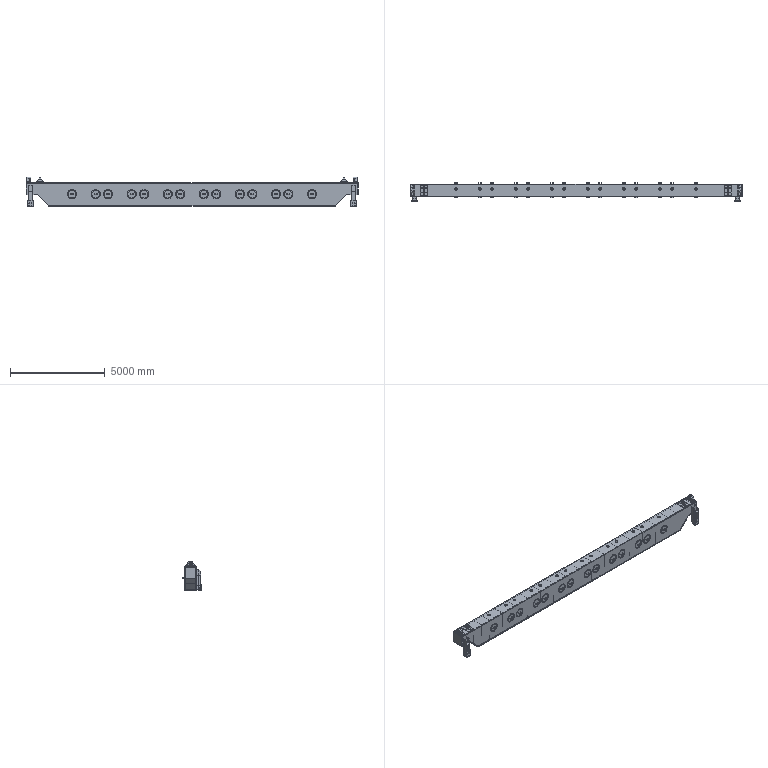Assembly | SolidWorks | mm | 127 component files | 127 solids | 2590 faces | box 17500 x 977 x 1565 mm | volume 2376243446 mm3 | cylinder 1510 | plane 840 | torus 224 | cone 16 | commonest cylinder face diameters 14 x252 5 x224 7 x224 26 x176 30 x168 40 x152 400 x56 55 x56
Bill of materials:
BearingHousing | 2 | Plain Carbon Steel | Prismatic block with both upper long edges chamfered, giving a six-sided end profile. A large round bore runs fully through, and there are small holes on the end face and the top face.
BearingHousingBasePlate | 2 | Plain Carbon Steel | Plain rectangular flat plate or bar with no visible holes or cutouts.
BearingHousingStiffener | 8 | Plain Carbon Steel | Extruded plate of uniform thickness with an irregular profile: a large angled cut along one side and a small chamfered corner, forming a gusset- or wedge-like shape.
ShaftBaffle | 4 | Plain Carbon Steel | Rectangular bar or flat link with two round through-holes, one near each end.
CoverHandle | 28 | Plain Carbon Steel | Hollow round tube bent into a U or handle shape: a straight middle run with roughly 90-degree radiused bends at both ends, which turn into short straight legs ending open.
RoundPlate | 28 | Plain Carbon Steel | Thin flat circular disc with four small holes evenly spaced near the outer edge.
ElectromagneticBeamBasePlate1 | 1 | Plain Carbon Steel | Long, narrow, thin strip with a row of repeated small hole clusters along its length.
ElectromagneticBeamBasePlate2 | 2 | Plain Carbon Steel | Thin, nearly square flat plate with two small rectangular notches cut into one edge.
ElectromagneticBeamBasePlate3 | 2 | Plain Carbon Steel | Thin flat rectangular plate with no visible holes or cutouts, shown in a tilted or oblique orientation.
ElectromagneticBeamEndPlate | 2 | Plain Carbon Steel | Plain rectangular flat plate of moderate thickness with no visible features.
ElectromagneticBeamRibPlate2 | 2 | Plain Carbon Steel | Thin rectangular plate with a centered rounded-corner rectangular cutout whose long axis follows the plate's long direction, forming a frame or bezel shape.
ElectromagneticBeamRibPlate3 | 2 | Plain Carbon Steel | Thin, nearly square plate with a centered rounded-corner rectangular through-cutout that is wider than it is tall.
ElectromagneticBeamTopPlate | 1 | Plain Carbon Steel | Long, thin, flat rectangular strip with a single row of 14 small round through-holes along its length: one single hole near each end and six evenly spaced pairs between them.
ElectromagneticBeamWeb | 2 | Plain Carbon Steel | Long, thin flat bar with a trapezoid-like outline. Short stepped tabs at each end, and the lower edge tapers inward at an angle at both ends. A single row of 14 round through-holes runs along the upper part, grouped as one single hole at each end with six pairs between them.
ElectromagneticMainBeamRibPlate1 | 17 | Plain Carbon Steel | Thin rectangular plate, taller than it is wide, with two rectangular through-cutouts with rounded corners, stacked vertically. The upper cutout is nearly square and the lower one is a taller rectangle.
Hanger | 2 | Plain Carbon Steel | Thick, flat lug or tab plate with a wide flat base, short vertical sides, sides that taper inward, and a rounded arched top. There is one round through-hole in the upper-central region.
HangerBasePlate | 2 | Plain Carbon Steel | Plain rectangular flat plate of uniform thickness with no visible holes, cutouts or edge features.
HangerStiffener | 8 | Plain Carbon Steel | Thick flat plate with a five-sided outline: a vertical left edge, a flat bottom edge, a long diagonal edge running from the top-left down to the right side, a short vertical right edge, and a small 45-degree-like chamfer at the bottom-left corner.
250I-beam | 2 | Plain Carbon Steel | Short H-section piece: two parallel flat flanges joined by a central web with filleted inner corners. The web ends partway along the length, so the two flanges continue as separate tabs. Each flange has chamfered corners at opposite ends and one round through-hole near the extended tab end.
250I-beamMountingPlate | 2 | Plain Carbon Steel | Rectangular flat plate, nearly square, with four obround (slotted) through-holes arranged in a 2x2 pattern. The slots are elongated horizontally in the face view.
250I-beamStiffener | 8 | Plain Carbon Steel | Rectangular flat plate of uniform thickness with both corners along one long edge chamfered.
Mates:
1. coincident | ElectromagneticBeamTopPlate-1 face at (-6575.465, 3561.733, 6674.043) dir (0, 0, -1) | ElectromagneticBeamWeb-1 face at (-6575.465, 2971.733, 6674.043) dir (0, 0, 1)
2. coincident | ElectromagneticBeamTopPlate-1 face at (-6575.465, 3561.733, 6674.043) dir (-1, 0, 0) | ElectromagneticBeamWeb-1 face at (-6575.465, 2971.733, 6094.043) dir (-1, 0, 0)
3. distance | ElectromagneticBeamTopPlate-1 face at (-6575.465, 2911.733, 6674.043) dir (0, -1, 0) | ElectromagneticBeamWeb-1 face at (-6575.465, 2931.733, 6674.043) dir (0, -1, 0)
4. coincident | ElectromagneticBeamTopPlate-1 face at (-6575.465, 3561.733, 6674.043) dir (0, 0, -1) | ElectromagneticBeamWeb-2 face at (-6575.465, 3541.733, 6674.043) dir (0, 0, 1)
5. coincident | ElectromagneticBeamTopPlate-1 face at (-6575.465, 3561.733, 6674.043) dir (-1, 0, 0) | ElectromagneticBeamWeb-2 face at (-6575.465, 3541.733, 6094.043) dir (-1, 0, 0)
6. distance | ElectromagneticBeamTopPlate-1 face at (-6575.465, 3561.733, 6674.043) dir (0, 1, 0) | ElectromagneticBeamWeb-2 face at (-6575.465, 3541.733, 6674.043) dir (0, 1, 0)
7. coincident | ElectromagneticBeamTopPlate-1 face at (-6575.465, 3561.733, 6674.043) dir (-1, 0, 0) | ElectromagneticBeamEndPlate-1 face at (-6575.465, 2911.733, 6074.043) dir (1, 0, 0)
8. coincident | ElectromagneticBeamTopPlate-1 face at (-6575.465, 3561.733, 6674.043) dir (0, 1, 0) | ElectromagneticBeamEndPlate-1 face at (-6575.465, 3561.733, 6074.043) dir (0, 1, 0)
9. coincident | ElectromagneticBeamTopPlate-1 face at (-6575.465, 3561.733, 6704.043) dir (0, 0, 1) | ElectromagneticBeamEndPlate-1 face at (-6575.465, 2911.733, 6704.043) dir (0, 0, 1)
10. coincident | ElectromagneticBeamWeb-1 face at (-5995.465, 2971.733, 6094.043) dir (0, 0, -1) | ElectromagneticBeamBasePlate2-1 face at (-6575.465, 3561.733, 6094.043) dir (0, 0, 1)
11. coincident | ElectromagneticBeamEndPlate-1 face at (-6575.465, 2911.733, 6074.043) dir (1, 0, 0) | ElectromagneticBeamBasePlate2-1 face at (-6575.465, 3561.733, 6074.043) dir (-1, 0, 0)
12. coincident | ElectromagneticBeamEndPlate-1 face at (-6575.465, 3561.733, 6074.043) dir (0, 1, 0) | ElectromagneticBeamBasePlate2-1 face at (-6575.465, 3561.733, 6074.043) dir (0, 1, 0)
13. coincident | ElectromagneticBeamWeb-1 face at (-5395.465, 2971.733, 5474.043) dir (-0.7186, 0, -0.6954) | ElectromagneticBeamBasePlate3-1 face at (-5395.465, 3561.733, 5474.043) dir (0.7186, 0, 0.6954)
14. coincident | ElectromagneticBeamBasePlate2-1 face at (-6237.465, 2911.733, 6074.043) dir (0, -1, 0) | ElectromagneticBeamBasePlate3-1 face at (-5409.837, 2911.733, 5460.135) dir (0, -1, 0)
15. coincident | ElectromagneticBeamWeb-1 edge at (-5395.465, 2971.733, 5474.043) dir (0, -1, 0) | ElectromagneticBeamBasePlate3-1 face at (-5409.837, 3561.733, 5460.135) dir (0.6954, 0, -0.7186)
16. coincident | ElectromagneticBeamWeb-1 face at (9684.535, 2971.733, 5474.043) dir (0, 0, -1) | ElectromagneticBeamBasePlate1-1 face at (-5395.465, 3561.733, 5474.043) dir (0, 0, 1)
17. coincident | ElectromagneticBeamBasePlate3-1 face at (-5409.837, 2911.733, 5460.135) dir (0, -1, 0) | ElectromagneticBeamBasePlate1-1 face at (-5395.465, 2911.733, 5444.043) dir (0, -1, 0)
18. coincident | ElectromagneticBeamBasePlate3-1 edge at (-5395.465, 2911.733, 5474.043) dir (0, 1, 0) | ElectromagneticBeamBasePlate1-1 face at (-5395.465, 3561.733, 5444.043) dir (-1, 0, 0)
19. coincident | ElectromagneticBeamWeb-2 face at (-6575.465, 3501.733, 6674.043) dir (0, -1, 0) | ElectromagneticMainBeamRibPlate1-1 face at (-4513.465, 3501.733, 6674.043) dir (0, 1, 0)
20. coincident | ElectromagneticBeamTopPlate-1 face at (-6575.465, 3561.733, 6674.043) dir (0, 0, -1) | ElectromagneticMainBeamRibPlate1-1 face at (-4513.465, 2971.733, 6674.043) dir (0, 0, 1)
21. distance | ElectromagneticBeamBasePlate1-1 face at (-4180.465, 3311.733, 5444.043) dir (0, 0, 1) r 45 | ElectromagneticMainBeamRibPlate1-1 face at (-4497.465, 2971.733, 6674.043) dir (1, 0, 0)
22. coincident | ElectromagneticBeamWeb-2 face at (-6575.465, 3501.733, 6674.043) dir (0, -1, 0) | ElectromagneticMainBeamRibPlate1-19 face at (-3563.465, 3501.733, 6674.043) dir (0, 1, 0)
23. coincident | ElectromagneticBeamTopPlate-1 face at (-6575.465, 3561.733, 6674.043) dir (0, 0, -1) | ElectromagneticMainBeamRibPlate1-19 face at (-3563.465, 2971.733, 6674.043) dir (0, 0, 1)
24. distance | ElectromagneticMainBeamRibPlate1-19 face at (-3563.465, 2971.733, 6674.043) dir (-1, 0, 0) | ElectromagneticBeamBasePlate1-1 face at (-4180.465, 3311.733, 5444.043) dir (0, 0, 1) r 45
25. coincident | ElectromagneticBeamWeb-2 face at (-6575.465, 3501.733, 6674.043) dir (0, -1, 0) | ElectromagneticMainBeamRibPlate1-22 face at (-2613.465, 3501.733, 6674.043) dir (0, 1, 0)
26. coincident | ElectromagneticBeamTopPlate-1 face at (-6575.465, 3561.733, 6674.043) dir (0, 0, -1) | ElectromagneticMainBeamRibPlate1-22 face at (-2613.465, 2971.733, 6674.043) dir (0, 0, 1)
27. distance | ElectromagneticMainBeamRibPlate1-22 face at (-2613.465, 2971.733, 6674.043) dir (-1, 0, 0) | ElectromagneticBeamBasePlate1-1 face at (-2930.465, 3311.733, 5444.043) dir (0, 0, 1) r 45
28. coincident | ElectromagneticBeamWeb-2 face at (-6575.465, 3501.733, 6674.043) dir (0, -1, 0) | ElectromagneticMainBeamRibPlate1-32 face at (2136.535, 3501.733, 6674.043) dir (0, 1, 0)
29. coincident | ElectromagneticBeamTopPlate-1 face at (-6575.465, 3561.733, 6674.043) dir (0, 0, -1) | ElectromagneticMainBeamRibPlate1-32 face at (2136.535, 2971.733, 6674.043) dir (0, 0, 1)
30. distance | ElectromagneticMainBeamRibPlate1-32 face at (2136.535, 2971.733, 6674.043) dir (-1, 0, 0) | ElectromagneticBeamBasePlate1-1 face at (1519.535, 3311.733, 5444.043) dir (0, 0, 1) r 45
31. coincident | ElectromagneticBeamWeb-2 face at (-6575.465, 3501.733, 6674.043) dir (0, -1, 0) | ElectromagneticBeamRibPlate2-1 face at (-5697.465, 3501.733, 5810.043) dir (0, 1, 0)
32. coincident | ElectromagneticBeamTopPlate-1 face at (-6575.465, 3561.733, 6674.043) dir (0, 0, -1) | ElectromagneticBeamRibPlate2-1 face at (-5697.465, 2971.733, 6674.043) dir (0, 0, 1)
33. distance | ElectromagneticMainBeamRibPlate1-16 face at (-5113.465, 2971.733, 6674.043) dir (-1, 0, 0) | ElectromagneticBeamRibPlate2-1 face at (-5713.465, 2971.733, 5810.043) dir (-1, 0, 0)
34. coincident | ElectromagneticBeamWeb-2 face at (-6575.465, 3501.733, 6674.043) dir (0, -1, 0) | ElectromagneticBeamRibPlate3-1 face at (-6297.465, 3501.733, 6094.043) dir (0, 1, 0)
35. coincident | ElectromagneticBeamTopPlate-1 face at (-6575.465, 3561.733, 6674.043) dir (0, 0, -1) | ElectromagneticBeamRibPlate3-1 face at (-6297.465, 2971.733, 6674.043) dir (0, 0, 1)
36. distance | ElectromagneticBeamRibPlate2-1 face at (-5713.465, 2971.733, 5810.043) dir (-1, 0, 0) | ElectromagneticBeamRibPlate3-1 face at (-6313.465, 2971.733, 6094.043) dir (-1, 0, 0)
37. coincident | ElectromagneticBeamTopPlate-1 face at (-6575.465, 3561.733, 6704.043) dir (0, 0, 1) | BearingHousing-1/BearingHousingBasePlate-1 face at (10654.535, 2961.733, 6704.043) dir (0, 0, -1)
38. distance | ElectromagneticBeamEndPlate-2 face at (10894.535, 2911.733, 6704.043) dir (1, 0, 0) | BearingHousing-1/BearingHousingBasePlate-1 face at (10854.535, 2961.733, 6704.043) dir (1, 0, 0)
39. distance | BearingHousing-1/BearingHousingBasePlate-1 face at (10654.535, 2961.733, 6704.043) dir (0, -1, 0) | ElectromagneticBeamTopPlate-1 face at (-6575.465, 2911.733, 6674.043) dir (0, -1, 0)
40. coincident | ElectromagneticBeamTopPlate-1 face at (-6575.465, 3561.733, 6704.043) dir (0, 0, 1) | Hanger-1/HangerBasePlate-1 face at (9974.535, 2961.733, 6704.043) dir (0, 0, -1)
41. distance | BearingHousing-1/BearingHousingBasePlate-1 face at (10854.535, 2961.733, 6704.043) dir (1, 0, 0) | Hanger-1/HangerBasePlate-1 face at (10354.535, 2961.733, 6704.043) dir (1, 0, 0)
42. coincident | BearingHousing-1/BearingHousingBasePlate-1 face at (10654.535, 3511.733, 6704.043) dir (0, 1, 0) | Hanger-1/HangerBasePlate-1 face at (9974.535, 3511.733, 6704.043) dir (0, 1, 0)
43. coincident | ElectromagneticBeamTopPlate-1 face at (-6575.465, 3561.733, 6704.043) dir (0, 0, 1) | BearingHousing-3/BearingHousingBasePlate-1 face at (-6365.465, 3511.733, 6704.043) dir (0, 0, -1)
44. distance | ElectromagneticBeamEndPlate-1 face at (-6605.465, 2911.733, 6074.043) dir (-1, 0, 0) | BearingHousing-3/BearingHousingBasePlate-1 face at (-6565.465, 3511.733, 6704.043) dir (-1, 0, 0)
45. coincident | ElectromagneticBeamTopPlate-1 face at (-6575.465, 3561.733, 6704.043) dir (0, 0, 1) | Hanger-3/HangerBasePlate-1 face at (-5685.465, 3511.733, 6704.043) dir (0, 0, -1)
46. distance | BearingHousing-3/BearingHousingBasePlate-1 face at (-6565.465, 3511.733, 6704.043) dir (-1, 0, 0) | Hanger-3/HangerBasePlate-1 face at (-6065.465, 3511.733, 6704.043) dir (-1, 0, 0)
47. coincident | BearingHousing-3/BearingHousingBasePlate-1 face at (-6365.465, 2961.733, 6704.043) dir (0, -1, 0) | Hanger-3/HangerBasePlate-1 face at (-5685.465, 2961.733, 6704.043) dir (0, -1, 0)
48. distance | BearingHousing-3/BearingHousingBasePlate-1 face at (-6365.465, 2961.733, 6704.043) dir (0, -1, 0) | ElectromagneticBeamTopPlate-1 face at (-6575.465, 2911.733, 6674.043) dir (0, -1, 0)
49. coincident | ElectromagneticBeamWeb-1 face at (-6575.465, 2931.733, 6674.043) dir (0, -1, 0) | WeldedI-beam-1/250I-beam-1 face at (-6497.465, 2931.733, 6524.043) dir (0, 1, 0)
50. distance | ElectromagneticBeamTopPlate-1 face at (-6575.465, 3561.733, 6704.043) dir (0, 0, 1) | WeldedI-beam-1/250I-beam-1 face at (-6274.465, 2789.233, 6524.043) dir (0, 0, 1)
51. coincident | ElectromagneticBeamBasePlate2-1 face at (-6497.465, 2911.733, 6074.043) dir (1, 0, 0) | WeldedI-beam-1/250I-beam-1 face at (-6497.465, 2681.733, 6524.043) dir (-1, 0, 0)
52. coincident | ElectromagneticBeamWeb-1 face at (-6575.465, 2931.733, 6674.043) dir (0, -1, 0) | CoverPlate-57/RoundPlate-1 face at (-4180.465, 2931.733, 6089.043) dir (0, 1, 0)
53. concentric | ElectromagneticBeamWeb-1 face at (-4180.465, 2971.733, 6089.043) dir (0, -1, 0) r 200 | CoverPlate-57/RoundPlate-1 face at (-4180.465, 2931.733, 6089.043) dir (0, -1, 0) r 250
54. parallel | ElectromagneticBeamTopPlate-1 face at (-6575.465, 3561.733, 6704.043) dir (0, 0, 1) | CoverPlate-57 plane at (-5270.021, 4189.28, 4936.162) dir (0, 0, 1)
55. coincident | ElectromagneticBeamWeb-2 face at (-6575.465, 3541.733, 6674.043) dir (0, 1, 0) | CoverPlate-85/RoundPlate-1 face at (-4180.465, 3541.733, 6089.043) dir (0, -1, 0)
56. concentric | ElectromagneticBeamWeb-2 face at (-4180.465, 3541.733, 6089.043) dir (0, -1, 0) r 200 | CoverPlate-85/RoundPlate-1 face at (-4180.465, 3541.733, 6089.043) dir (0, 1, 0) r 250
57. parallel | ElectromagneticBeamTopPlate-1 face at (-6575.465, 3561.733, 6704.043) dir (0, 0, 1) | CoverPlate-85 plane at (-5270.021, 2284.186, 7241.924) dir (0, 0, -1)
58. coincident | ElectromagneticBeamBasePlate2-2 face at (10786.535, 2911.733, 6094.043) dir (-1, 0, 0) | WeldedI-beam-2/250I-beam-1 face at (10786.535, 2931.733, 6524.043) dir (1, 0, 0)
59. coincident | ElectromagneticBeamWeb-1 face at (-6575.465, 2931.733, 6674.043) dir (0, -1, 0) | WeldedI-beam-2/250I-beam-1 face at (10772.535, 2931.733, 6524.043) dir (0, 1, 0)
60. distance | ElectromagneticBeamTopPlate-1 face at (-6575.465, 3561.733, 6704.043) dir (0, 0, 1) | WeldedI-beam-2/250I-beam-1 face at (10759.535, 2789.233, 6524.043) dir (0, 0, 1)
61. coincident | BearingHousingBasePlate-1 face at (818.518, 1208.13, 1203.354) dir (0, 0, 1) | BearingHousing-1 face at (968.518, 1208.13, 1203.354) dir (0, 0, -1)
62. coincident | BearingHousingBasePlate-1 face at (818.518, 1008.13, 1173.354) dir (0, -1, 0) | BearingHousing-1 face at (968.518, 1008.13, 1203.354) dir (0, -1, 0)
63. distance | BearingHousing-1 face at (968.518, 1208.13, 1203.354) dir (-1, 0, 0) | BearingHousingBasePlate-1 face at (818.518, 1208.13, 1173.354) dir (-1, 0, 0)
64. coincident | BearingHousing-1 face at (1218.518, 1208.13, 1203.354) dir (1, 0, 0) | BearingHousingStiffener-1 face at (1218.518, 1158.13, 1228.354) dir (-1, 0, 0)
65. coincident | BearingHousingBasePlate-1 face at (818.518, 1208.13, 1203.354) dir (0, 0, 1) | BearingHousingStiffener-1 face at (1368.518, 1158.13, 1203.354) dir (0, 0, -1)
66. distance | BearingHousingBasePlate-1 face at (818.518, 1208.13, 1173.354) dir (0, 1, 0) | BearingHousingStiffener-1 face at (1368.518, 1188.13, 1203.354) dir (0, 1, 0)
67. coincident | BearingHousing-1 face at (1218.518, 1208.13, 1203.354) dir (1, 0, 0) | BearingHousingStiffener-2 face at (1218.518, 1028.13, 1228.354) dir (-1, 0, 0)
68. coincident | BearingHousingBasePlate-1 face at (818.518, 1208.13, 1203.354) dir (0, 0, 1) | BearingHousingStiffener-2 face at (1368.518, 1028.13, 1203.354) dir (0, 0, -1)
69. distance | BearingHousingStiffener-2 face at (1368.518, 1028.13, 1203.354) dir (0, -1, 0) | BearingHousingBasePlate-1 face at (818.518, 1008.13, 1173.354) dir (0, -1, 0)
70. coincident | BearingHousing-1 face at (968.518, 1008.13, 1203.354) dir (0, -1, 0) | ShaftBaffle-1 face at (1033.518, 1008.13, 1394.354) dir (0, 1, 0)
71. coincident | BearingHousing-1 face at (968.518, 1208.13, 1203.354) dir (0, 1, 0) | ShaftBaffle-2 face at (1033.518, 1208.13, 1397.354) dir (0, -1, 0)
72. concentric | BearingHousing-1 face at (1138.518, 1208.13, 1414.854) dir (0, 1, 0) r 5.1 | ShaftBaffle-2 face at (1138.518, 1208.13, 1414.854) dir (0, 1, 0) r 6.75
73. concentric | BearingHousing-1 face at (1048.518, 1208.13, 1414.854) dir (0, 1, 0) r 5.1 | ShaftBaffle-2 face at (1048.518, 1208.13, 1414.854) dir (0, 1, 0) r 6.75
74. concentric | BearingHousing-1 face at (1048.518, 1008.13, 1411.854) dir (0, -1, 0) r 5.1 | ShaftBaffle-1 face at (1048.518, 1000.13, 1411.854) dir (0, 1, 0) r 6.75
75. concentric | BearingHousing-1 face at (1138.518, 1008.13, 1411.854) dir (0, -1, 0) r 5.1 | ShaftBaffle-1 face at (1138.518, 1000.13, 1411.854) dir (0, 1, 0) r 6.75
76. coincident | RoundPlate-1 face at (1089.556, 1152.881, 1259.547) dir (0, 0, 1) | CoverHandle-1 face at (1164.556, 1152.881, 1259.547) dir (0, 0, -1)
77. coincident | RoundPlate-1 plane at (1089.556, 1152.881, 1259.547) dir (0, -1, 0) | CoverHandle-1 plane at (1014.556, 1152.881, 1259.547) dir (0, -1, 0)
78. distance | RoundPlate-1 plane at (1089.556, 1152.881, 1259.547) dir (1, 0, 0) | CoverHandle-1 plane at (1014.556, 1152.881, 1259.547) dir (1, 0, 0)
79. coincident | HangerBasePlate-1 face at (872.891, 1303.867, 1233.229) dir (0, 0, 1) | Hanger-1 face at (947.891, 1073.867, 1233.229) dir (0, 0, -1)
80. distance | Hanger-1 face at (1347.891, 1073.867, 1283.229) dir (1, 0, 0) | HangerBasePlate-1 face at (1422.891, 1303.867, 1203.229) dir (1, 0, 0)
81. distance | Hanger-1 face at (1147.891, 1073.867, 1358.229) dir (0, -1, 0) | HangerBasePlate-1 face at (872.891, 923.867, 1203.229) dir (0, -1, 0)
82. coincident | Hanger-1 face at (1147.891, 1073.867, 1358.229) dir (0, -1, 0) | HangerStiffener-1 face at (1047.891, 1073.867, 1383.229) dir (0, 1, 0)
83. coincident | HangerBasePlate-1 face at (872.891, 1303.867, 1233.229) dir (0, 0, 1) | HangerStiffener-1 face at (1047.891, 1048.867, 1233.229) dir (0, 0, -1)
84. distance | HangerStiffener-1 face at (1017.891, 1073.867, 1383.229) dir (-1, 0, 0) | Hanger-1 face at (947.891, 1073.867, 1283.229) dir (-1, 0, 0)
85. coincident | Hanger-1 face at (1147.891, 1073.867, 1358.229) dir (0, -1, 0) | HangerStiffener-2 face at (1277.891, 1073.867, 1383.229) dir (0, 1, 0)
86. coincident | HangerBasePlate-1 face at (872.891, 1303.867, 1233.229) dir (0, 0, 1) | HangerStiffener-2 face at (1277.891, 1048.867, 1233.229) dir (0, 0, -1)
87. distance | Hanger-1 face at (1347.891, 1073.867, 1283.229) dir (1, 0, 0) | HangerStiffener-2 face at (1277.891, 1073.867, 1383.229) dir (1, 0, 0)
88. coincident | 250I-beam-1 face at (1120.365, 1154.619, 1839.04) dir (0, -1, 0) | 250I-beamMountingPlate-1 face at (1081.365, 1154.619, 739.04) dir (0, 1, 0)
89. coincident | 250I-beam-1 face at (1329.365, 1262.119, 739.04) dir (0, 0, -1) | 250I-beamMountingPlate-1 face at (1081.365, 1134.619, 739.04) dir (0, 0, -1)
90. distance | 250I-beam-1 face at (1106.365, 1154.619, 1839.04) dir (-1, 0, 0) | 250I-beamMountingPlate-1 face at (1081.365, 1134.619, 739.04) dir (-1, 0, 0)
91. coincident | 250I-beam-1 face at (1342.365, 1154.619, 1839.04) dir (-1, 0, 0) | 250I-beamStiffener-1 face at (1342.365, 1404.619, 1523.04) dir (1, 0, 0)
92. coincident | 250I-beam-1 face at (1133.365, 1284.119, 1839.04) dir (0, 1, 0) | 250I-beamStiffener-1 face at (1133.865, 1284.119, 1523.04) dir (0, -1, 0)
93. distance | 250I-beam-1 face at (1329.365, 1262.119, 1839.04) dir (0, 0, 1) | 250I-beamStiffener-1 face at (1120.365, 1404.619, 1539.04) dir (0, 0, 1)
94. coincident | 250I-beam-1 face at (1120.365, 1262.119, 1839.04) dir (1, 0, 0) | 250I-beamStiffener-4 face at (1120.365, 1154.619, 1539.04) dir (-1, 0, 0)
95. coincident | 250I-beam-1 face at (1329.365, 1275.119, 1839.04) dir (0, -1, 0) | 250I-beamStiffener-4 face at (1133.865, 1275.119, 1539.04) dir (0, 1, 0)
96. coincident | 250I-beamStiffener-1 face at (1120.365, 1404.619, 1539.04) dir (0, 0, 1) | 250I-beamStiffener-4 face at (1120.365, 1154.619, 1539.04) dir (0, 0, 1)